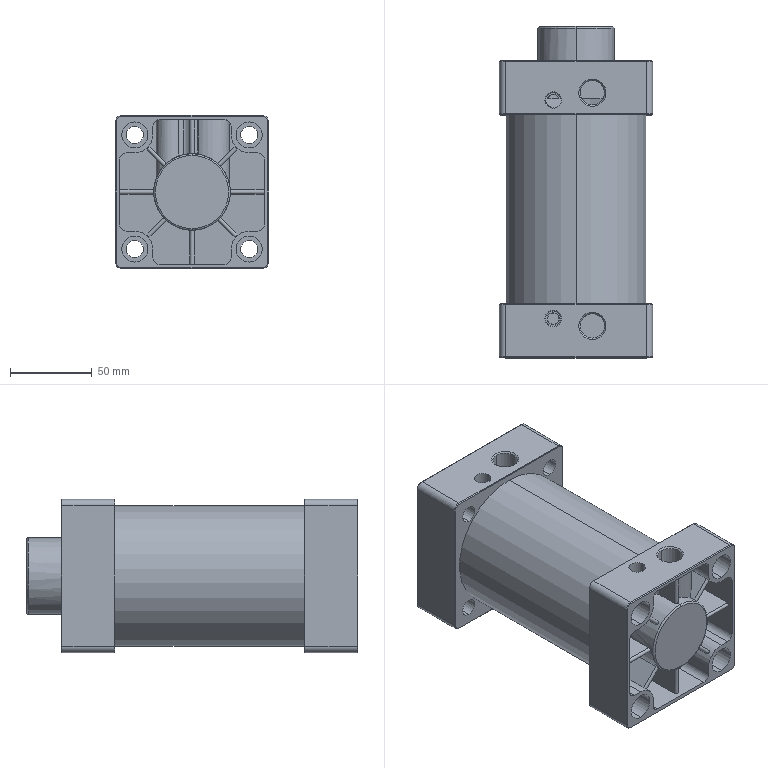Component | SolidWorks | AirTACCylinderFSC_80x75_S_FB-1_FSC_80x75_S_FB_0_c-1 | 1 solid | 298 faces | volume 369258 mm3 | cylinder 133 | plane 128 | cone 29 | torus 8 | commonest cylinder face diameters 8 x27 16 x21 2.5 x18 10.5 x16 22 x8 26 x5 36.4 x4 9.188 x4